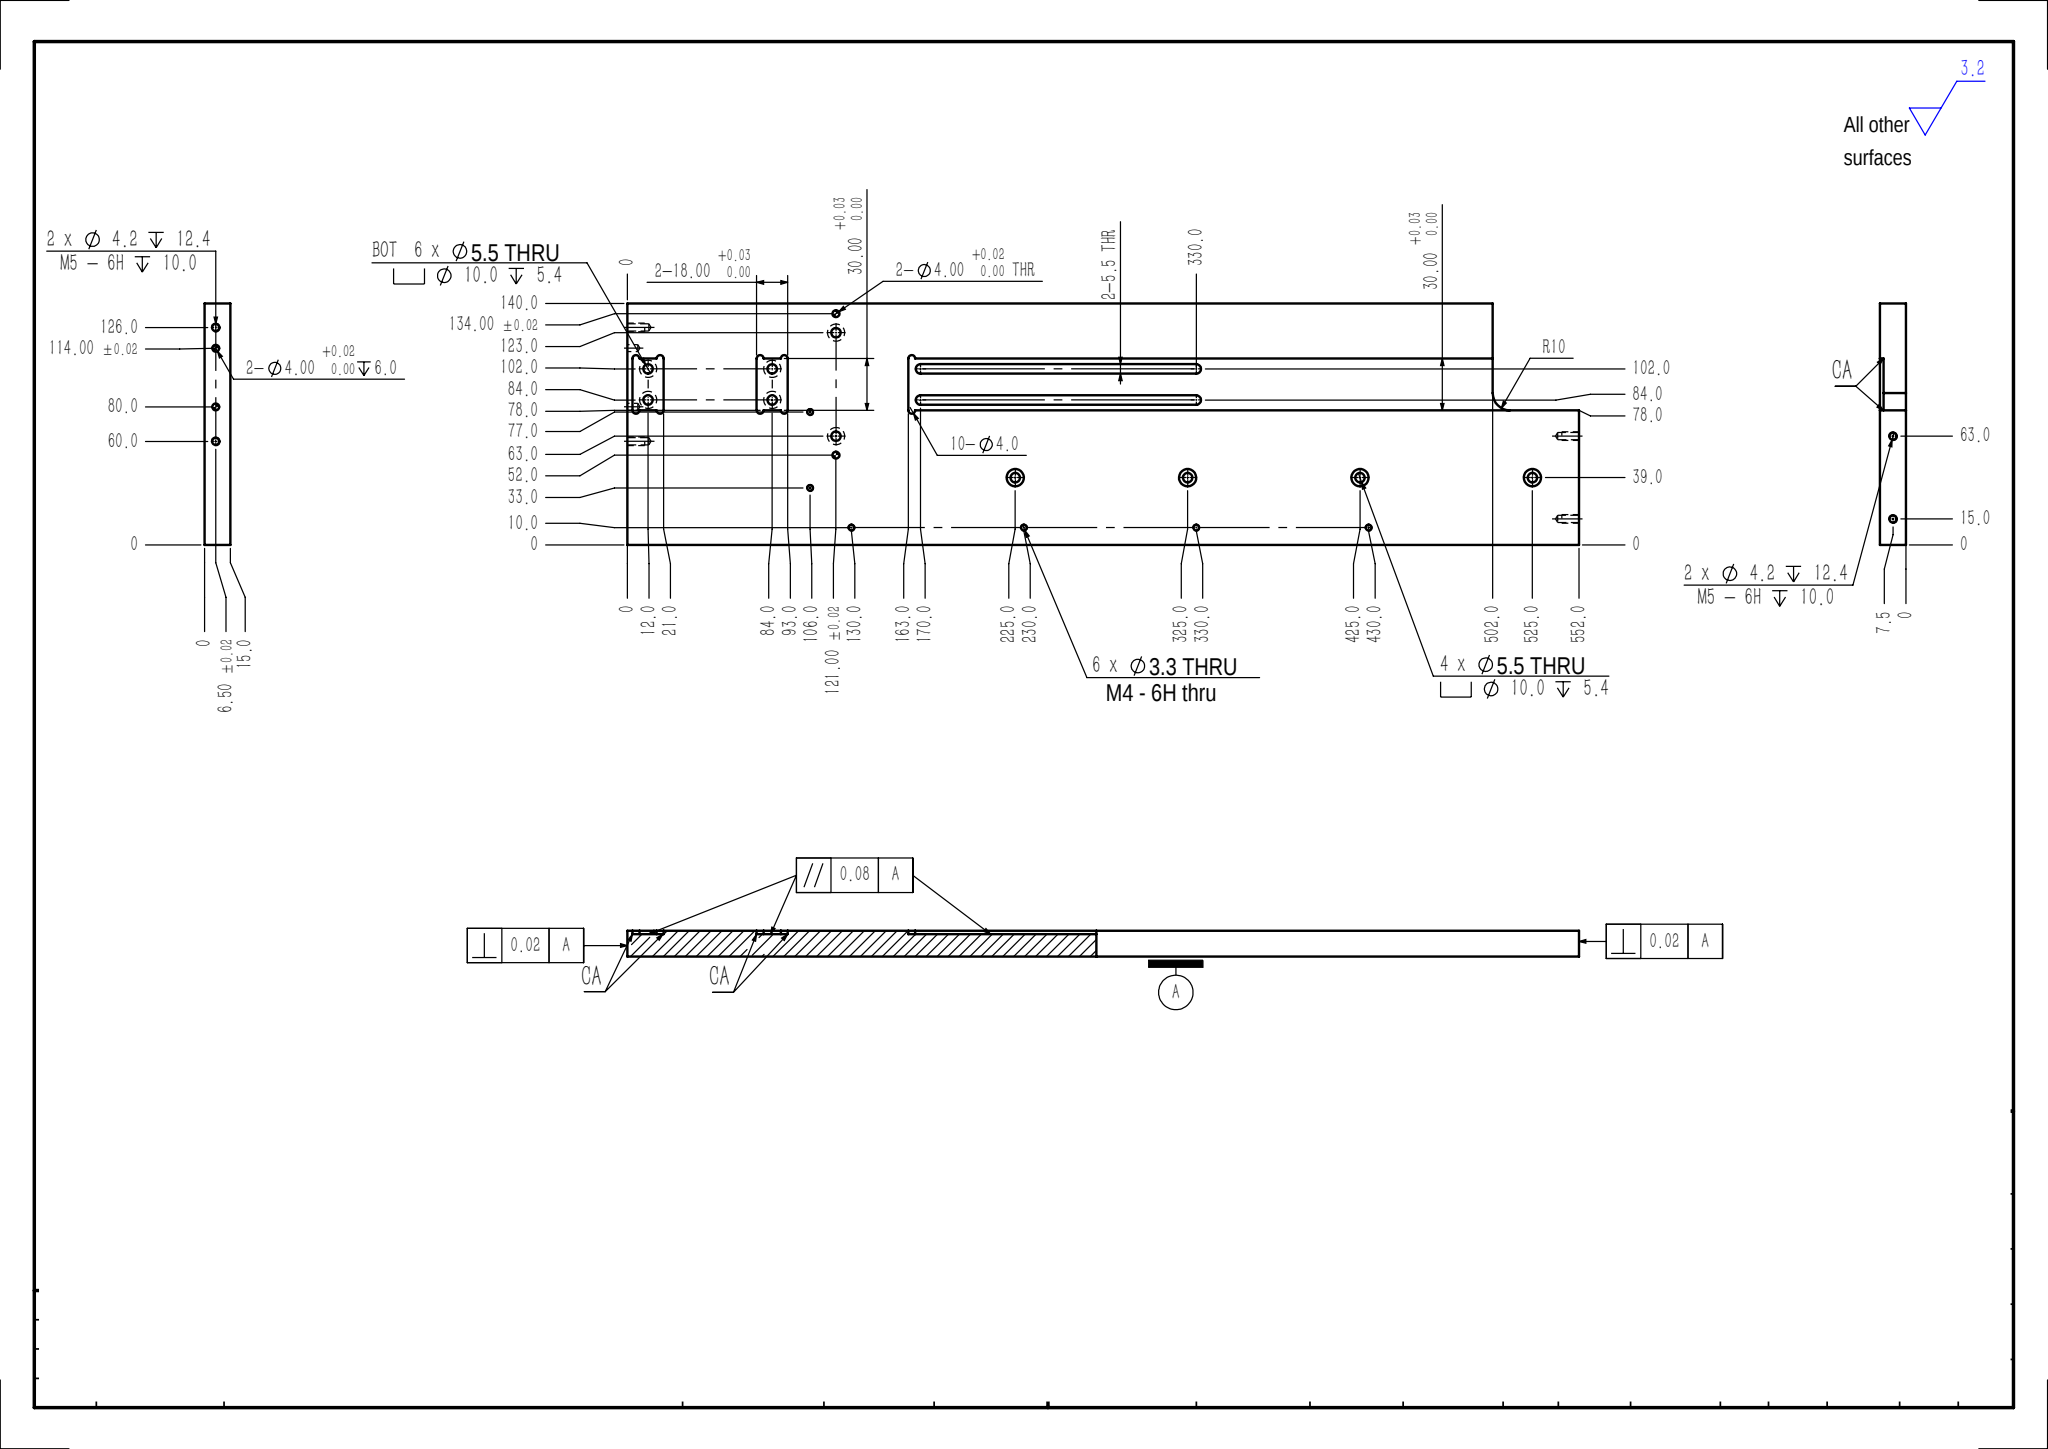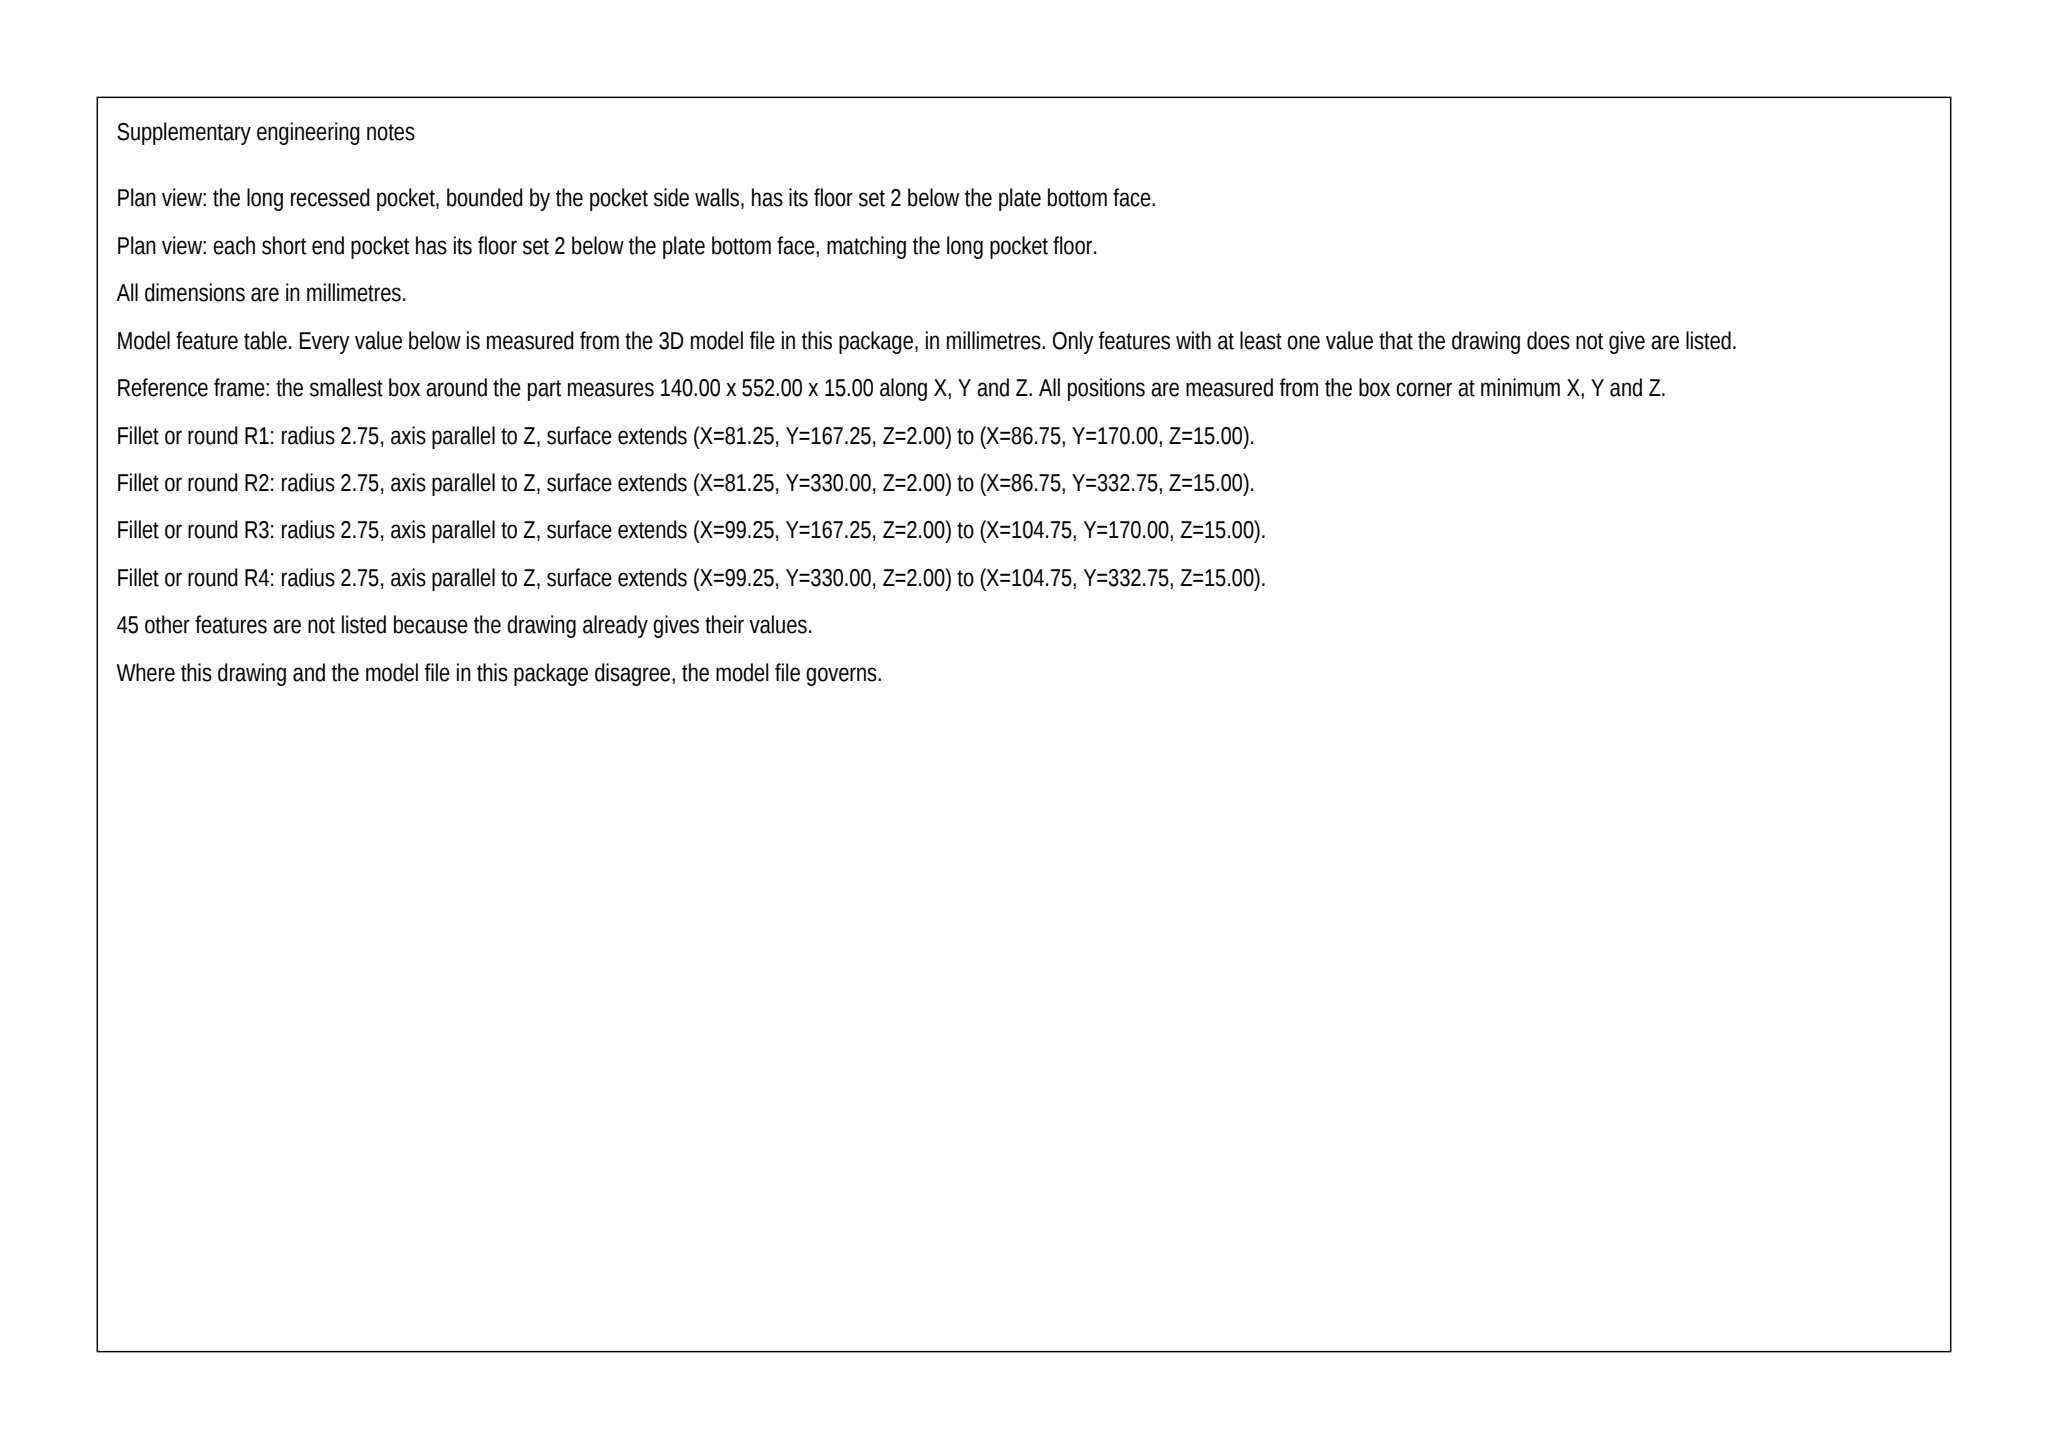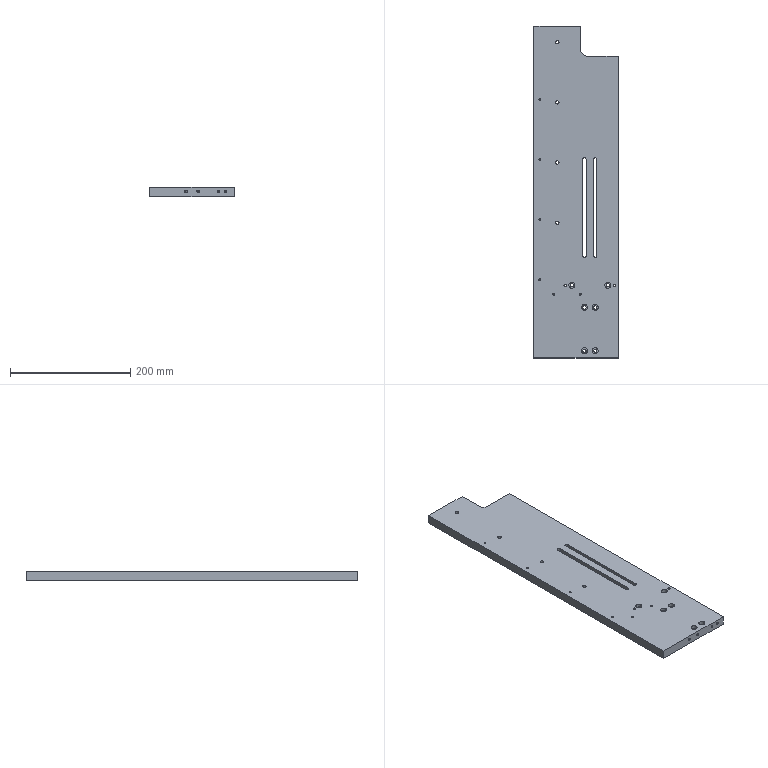Part | SolidWorks | mm | 1 solid | 135 faces | box 140 x 552 x 15 mm | volume 1058506 mm3 | cylinder 88 | plane 35 | cone 12 | commonest cylinder face diameters 5.5 x24 4 x23 10 x20 3.3 x12 4.2 x8 20 x1
build123d program:
from build123d import *

# Parameters (mm, degrees)
SKETCH1_W                                       = 140
SKETCH1_H                                       = 552
BOSS_EXTRUDE1_DEPTH                             = 7.5
SKETCH2_W                                       = 30
SKETCH2_H                                       = 18
SKETCH2_H_2                                     = 389
CUT_EXTRUDE1_DEPTH                              = 2
SKETCH3_R                                       = 2
CUT_EXTRUDE2_DEPTH                              = 2
M5_TAPPED_HOLE1_D                               = 4.2
M5_TAPPED_HOLE1_DEPTH                           = 12.4
M5_TAPPED_HOLE1_TIP                             = 1.262
M4_TAPPED_HOLE1_D                               = 3.3
M5_TAPPED_HOLE2_D                               = 4.2
M5_TAPPED_HOLE2_DEPTH                           = 12.4
M5_TAPPED_HOLE2_TIP                             = 1.262
SIZE_MM_DOWEL_PIN_HOLE2_D                       = 4
SIZE_MM_DOWEL_PIN_HOLE2_DEPTH                   = 6
SIZE_MM_DOWEL_PIN_HOLE2_TIP                     = 1.202
M5_HEX_SOCKET_HEAD_CAP_SCREW_CBORE1_D           = 5.5
M5_HEX_SOCKET_HEAD_CAP_SCREW_CBORE1_CBORE_D     = 10
M5_HEX_SOCKET_HEAD_CAP_SCREW_CBORE1_CBORE_DEPTH = 5.4
CUT_EXTRUDE3_DEPTH                              = 286.133
M4_TAPPED_HOLE2_D                               = 3.3
M5_HEX_SOCKET_HEAD_CAP_SCREW_CBORE2_D           = 5.5
M5_HEX_SOCKET_HEAD_CAP_SCREW_CBORE2_CBORE_D     = 10
M5_HEX_SOCKET_HEAD_CAP_SCREW_CBORE2_CBORE_DEPTH = 5.4
SIZE_MM_DOWEL_PIN_HOLE2_2_D                     = 4
CUT_EXTRUDE4_DEPTH                              = 286.133
M5_HEX_SOCKET_HEAD_CAP_SCREW_CBORE3_D           = 5.5
M5_HEX_SOCKET_HEAD_CAP_SCREW_CBORE3_CBORE_D     = 10
M5_HEX_SOCKET_HEAD_CAP_SCREW_CBORE3_CBORE_DEPTH = 5.4


with BuildPart() as part:
    # Sketch1 → Boss-Extrude1 (new, symmetric)
    with BuildSketch(Plane.XY):
        Rectangle(SKETCH1_W, SKETCH1_H)
    extrude(amount=BOSS_EXTRUDE1_DEPTH, both=True)

    # Sketch2 → Cut-Extrude1 (cut)
    with BuildSketch(Plane(origin=(0, 0, -7.5), x_dir=(-1, 0, 0), z_dir=(0, 0, -1))):
        with Locations((-23, -264)):
            Rectangle(SKETCH2_W, SKETCH2_H)
        with Locations((-23, -192)):
            Rectangle(SKETCH2_W, SKETCH2_H)
        with Locations((-23, 81.5)):
            Rectangle(SKETCH2_W, SKETCH2_H_2)
    extrude(amount=-CUT_EXTRUDE1_DEPTH, mode=Mode.SUBTRACT)

    # Sketch3 → Cut-Extrude2 (cut)
    with BuildSketch(Plane(origin=(0, 0, -7.5), x_dir=(-1, 0, 0), z_dir=(0, 0, -1))):
        with Locations((-8, -271)):
            Circle(SKETCH3_R)
        with Locations((-38, -271)):
            Circle(SKETCH3_R)
        with Locations((-8, -257)):
            Circle(SKETCH3_R)
        with Locations((-38, -257)):
            Circle(SKETCH3_R)
        with Locations((-8, -199)):
            Circle(SKETCH3_R)
        with Locations((-38, -199)):
            Circle(SKETCH3_R)
        with Locations((-8, -185)):
            Circle(SKETCH3_R)
        with Locations((-38, -185)):
            Circle(SKETCH3_R)
        with Locations((-8, -111)):
            Circle(SKETCH3_R)
        with Locations((-38, -111)):
            Circle(SKETCH3_R)
    extrude(amount=-CUT_EXTRUDE2_DEPTH, mode=Mode.SUBTRACT)

    # M5 Tapped Hole1
    with Locations(Plane(origin=(0, 276, 0), x_dir=(1, 0, 0), z_dir=(0, 1, 0))):
        with Locations((-7, 0), (-55, 0)):
            Hole(M5_TAPPED_HOLE1_D / 2, depth=M5_TAPPED_HOLE1_DEPTH)
            with Locations((0, 0, -(M5_TAPPED_HOLE1_DEPTH + M5_TAPPED_HOLE1_TIP / 2))):  # 118° drill point
                Cone(0, M5_TAPPED_HOLE1_D / 2, M5_TAPPED_HOLE1_TIP, mode=Mode.SUBTRACT)

    # M4 Tapped Hole1 (through all)
    with Locations(Plane.XY.offset(7.5)):
        with Locations((7, -170), (-37, -170)):
            Hole(M4_TAPPED_HOLE1_D / 2)

    # M5 Tapped Hole2
    with Locations(Plane(origin=(0, -276, 0), x_dir=(-1, 0, 0), z_dir=(0, -1, 0))):
        with Locations((-56, -1), (10, -1)):
            Hole(M5_TAPPED_HOLE2_D / 2, depth=M5_TAPPED_HOLE2_DEPTH)
            with Locations((0, 0, -(M5_TAPPED_HOLE2_DEPTH + M5_TAPPED_HOLE2_TIP / 2))):  # 118° drill point
                Cone(0, M5_TAPPED_HOLE2_D / 2, M5_TAPPED_HOLE2_TIP, mode=Mode.SUBTRACT)

    # Size mm Dowel Pin Hole2
    with Locations(Plane(origin=(0, -276, 0), x_dir=(-1, 0, 0), z_dir=(0, -1, 0))):
        with Locations((-44, -1), (-10, -1)):
            Hole(SIZE_MM_DOWEL_PIN_HOLE2_D / 2, depth=SIZE_MM_DOWEL_PIN_HOLE2_DEPTH)
            with Locations((0, 0, -(SIZE_MM_DOWEL_PIN_HOLE2_DEPTH + SIZE_MM_DOWEL_PIN_HOLE2_TIP / 2))):  # 118° drill point
                Cone(0, SIZE_MM_DOWEL_PIN_HOLE2_D / 2, SIZE_MM_DOWEL_PIN_HOLE2_TIP, mode=Mode.SUBTRACT)

    # M5 Hex Socket Head Cap Screw CBORE1 (through all)
    with Locations(Plane.XY.offset(7.5)):
        with Locations((32, -264), (14, -264), (32, -192), (14, -192)):
            CounterBoreHole(M5_HEX_SOCKET_HEAD_CAP_SCREW_CBORE1_D / 2, M5_HEX_SOCKET_HEAD_CAP_SCREW_CBORE1_CBORE_D / 2, M5_HEX_SOCKET_HEAD_CAP_SCREW_CBORE1_CBORE_DEPTH)

    # Sketch21 → Cut-Extrude3 (cut, through all)
    with BuildSketch(Plane.XY.offset(7.5)):
        with BuildLine():
            Line((29.25, -106), (29.25, 54))
            ThreePointArc((29.25, 54), (32, 56.75), (34.75, 54))
            Line((34.75, 54), (34.75, -106))
            ThreePointArc((34.75, -106), (32, -108.75), (29.25, -106))
        make_face()
        with BuildLine():
            Line((16.75, -106), (16.75, 54))
            ThreePointArc((16.75, 54), (14, 56.75), (11.25, 54))
            Line((11.25, 54), (11.25, -106))
            ThreePointArc((11.25, -106), (14, -108.75), (16.75, -106))
        make_face()
    extrude(amount=-CUT_EXTRUDE3_DEPTH, mode=Mode.SUBTRACT)

    # M4 Tapped Hole2 (through all)
    with Locations(Plane.XY.offset(7.5)):
        with Locations((-60, -146), (-60, -46), (-60, 54), (-60, 154)):
            Hole(M4_TAPPED_HOLE2_D / 2)

    # M5 Hex Socket Head Cap Screw CBORE2 (through all)
    with Locations(Plane.XY.offset(7.5)):
        with Locations((53, -155), (-7, -155)):
            CounterBoreHole(M5_HEX_SOCKET_HEAD_CAP_SCREW_CBORE2_D / 2, M5_HEX_SOCKET_HEAD_CAP_SCREW_CBORE2_CBORE_D / 2, M5_HEX_SOCKET_HEAD_CAP_SCREW_CBORE2_CBORE_DEPTH)

    # Size mm Dowel Pin Hole2_2 (through all)
    with Locations(Plane.XY.offset(7.5)):
        with Locations((64, -155), (-18, -155)):
            Hole(SIZE_MM_DOWEL_PIN_HOLE2_2_D / 2)

    # Sketch31 → Cut-Extrude4 (cut, through all)
    with BuildSketch(Plane(origin=(0, 0, -7.5), x_dir=(-1, 0, 0), z_dir=(0, 0, -1))):
        with BuildLine():
            Line((-70, 276), (-8, 276))
            Line((-8, 276), (-8, 236))
            ThreePointArc((-8, 236), (-10.929, 228.929), (-18, 226))
            Line((-18, 226), (-70, 226))
            Line((-70, 226), (-70, 276))
        make_face()
    extrude(amount=-CUT_EXTRUDE4_DEPTH, mode=Mode.SUBTRACT)

    # M5 Hex Socket Head Cap Screw CBORE3 (through all)
    with Locations(Plane(origin=(0, 0, -7.5), x_dir=(-1, 0, 0), z_dir=(0, 0, -1))):
        with Locations((31, -51), (31, 49), (31, 149), (31, 249)):
            CounterBoreHole(M5_HEX_SOCKET_HEAD_CAP_SCREW_CBORE3_D / 2, M5_HEX_SOCKET_HEAD_CAP_SCREW_CBORE3_CBORE_D / 2, M5_HEX_SOCKET_HEAD_CAP_SCREW_CBORE3_CBORE_DEPTH)


solid = part.part